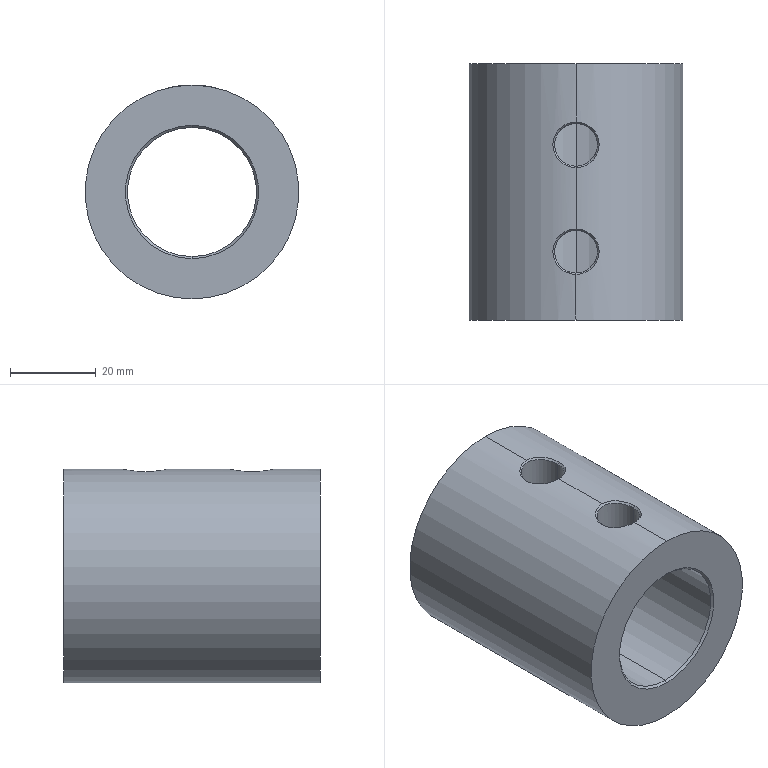Component | SolidWorks | 01-01Chassis-1_01-01-05ChassisWeldment5-2 | 1 solid | 22 faces | volume 73227 mm3 | spline 8 | cylinder 8 | cone 4 | plane 2 | commonest cylinder face diameters 10 x4 30.2 x2 50 x2 | material 45